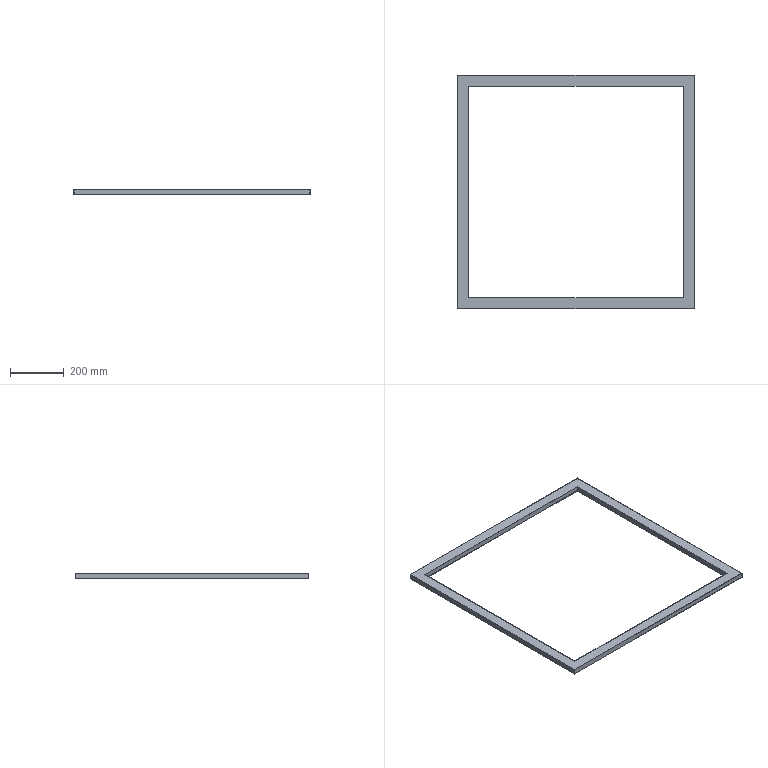Component | SolidWorks | 200TonPunchPress3DDrawing.sldasm-Part-1-1 | 1 solid | 20 faces | box 882 x 870 x 20 mm | volume 749056 mm3 | plane 20
STEP:
#1=COLOUR_RGB('',0.7922,0.8196,0.9333);
#2=FILL_AREA_STYLE_COLOUR('',#1);
#3=FILL_AREA_STYLE('',(#2));
#4=SURFACE_STYLE_FILL_AREA(#3);
#5=SURFACE_SIDE_STYLE('',(#4));
#6=SURFACE_STYLE_USAGE(.BOTH.,#5);
#7=PRESENTATION_STYLE_ASSIGNMENT((#6));
#8=CARTESIAN_POINT('',(-15.827,-41.278,51.26));
#9=VERTEX_POINT('',#8);
#10=CARTESIAN_POINT('',(15.906,-41.278,51.26));
#11=VERTEX_POINT('',#10);
#12=CARTESIAN_POINT('',(-20.057,-41.278,51.26));
#13=DIRECTION('',(1.,-0.,0.));
#14=VECTOR('',#13,39.37);
#15=LINE('',#12,#14);
#16=EDGE_CURVE('',#9,#11,#15,.T.);
#17=ORIENTED_EDGE('',*,*,#16,.T.);
#18=CARTESIAN_POINT('',(15.906,-41.278,51.89));
#19=VERTEX_POINT('',#18);
#20=CARTESIAN_POINT('',(15.906,-41.278,51.89));
#21=DIRECTION('',(0.,0.,1.));
#22=VECTOR('',#21,39.37);
#23=LINE('',#20,#22);
#24=EDGE_CURVE('',#11,#19,#23,.T.);
#25=ORIENTED_EDGE('',*,*,#24,.T.);
#26=CARTESIAN_POINT('',(-15.827,-41.278,51.89));
#27=VERTEX_POINT('',#26);
#28=CARTESIAN_POINT('',(-20.057,-41.278,51.89));
#29=DIRECTION('',(1.,-0.,0.));
#30=VECTOR('',#29,39.37);
#31=LINE('',#28,#30);
#32=EDGE_CURVE('',#27,#19,#31,.T.);
#33=ORIENTED_EDGE('',*,*,#32,.F.);
#34=CARTESIAN_POINT('',(-15.827,-41.278,51.89));
#35=DIRECTION('',(0.,0.,-1.));
#36=VECTOR('',#35,39.37);
#37=LINE('',#34,#36);
#38=EDGE_CURVE('',#27,#9,#37,.T.);
#39=ORIENTED_EDGE('',*,*,#38,.T.);
#40=EDGE_LOOP('',(#17,#25,#33,#39));
#41=FACE_OUTER_BOUND('',#40,.T.);
#42=CARTESIAN_POINT('',(-20.057,-41.278,51.89));
#43=DIRECTION('',(-0.,-1.,0.));
#44=DIRECTION('',(-1.,0.,0.));
#45=AXIS2_PLACEMENT_3D('',#42,#43,#44);
#46=PLANE('',#45);
#47=ADVANCED_FACE('',(#41),#46,.T.);
#48=CARTESIAN_POINT('',(15.906,-72.538,51.89));
#49=VERTEX_POINT('',#48);
#50=CARTESIAN_POINT('',(15.906,-72.538,51.89));
#51=DIRECTION('',(0.,1.,0.));
#52=VECTOR('',#51,39.37);
#53=LINE('',#50,#52);
#54=EDGE_CURVE('',#49,#19,#53,.T.);
#55=ORIENTED_EDGE('',*,*,#54,.F.);
#56=CARTESIAN_POINT('',(-15.827,-72.538,51.89));
#57=VERTEX_POINT('',#56);
#58=CARTESIAN_POINT('',(-15.827,-72.538,51.89));
#59=DIRECTION('',(1.,-0.,0.));
#60=VECTOR('',#59,39.37);
#61=LINE('',#58,#60);
#62=EDGE_CURVE('',#57,#49,#61,.T.);
#63=ORIENTED_EDGE('',*,*,#62,.F.);
#64=CARTESIAN_POINT('',(-15.827,-41.278,51.89));
#65=DIRECTION('',(0.,-1.,0.));
#66=VECTOR('',#65,39.37);
#67=LINE('',#64,#66);
#68=EDGE_CURVE('',#27,#57,#67,.T.);
#69=ORIENTED_EDGE('',*,*,#68,.F.);
#70=ORIENTED_EDGE('',*,*,#32,.T.);
#71=EDGE_LOOP('',(#55,#63,#69,#70));
#72=FACE_BOUND('',#71,.T.);
#73=CARTESIAN_POINT('',(-17.244,-73.955,51.89));
#74=VERTEX_POINT('',#73);
#75=CARTESIAN_POINT('',(17.323,-73.955,51.89));
#76=VERTEX_POINT('',#75);
#77=CARTESIAN_POINT('',(-17.244,-73.955,51.89));
#78=DIRECTION('',(1.,-0.,0.));
#79=VECTOR('',#78,39.37);
#80=LINE('',#77,#79);
#81=EDGE_CURVE('',#74,#76,#80,.T.);
#82=ORIENTED_EDGE('',*,*,#81,.T.);
#83=CARTESIAN_POINT('',(17.323,-39.86,51.89));
#84=VERTEX_POINT('',#83);
#85=CARTESIAN_POINT('',(17.323,-73.955,51.89));
#86=DIRECTION('',(0.,1.,0.));
#87=VECTOR('',#86,39.37);
#88=LINE('',#85,#87);
#89=EDGE_CURVE('',#76,#84,#88,.T.);
#90=ORIENTED_EDGE('',*,*,#89,.T.);
#91=CARTESIAN_POINT('',(-17.244,-39.86,51.89));
#92=VERTEX_POINT('',#91);
#93=CARTESIAN_POINT('',(-20.057,-39.86,51.89));
#94=DIRECTION('',(1.,-0.,0.));
#95=VECTOR('',#94,39.37);
#96=LINE('',#93,#95);
#97=EDGE_CURVE('',#92,#84,#96,.T.);
#98=ORIENTED_EDGE('',*,*,#97,.F.);
#99=CARTESIAN_POINT('',(-17.244,-39.86,51.89));
#100=DIRECTION('',(0.,-1.,0.));
#101=VECTOR('',#100,39.37);
#102=LINE('',#99,#101);
#103=EDGE_CURVE('',#92,#74,#102,.T.);
#104=ORIENTED_EDGE('',*,*,#103,.T.);
#105=EDGE_LOOP('',(#82,#90,#98,#104));
#106=FACE_OUTER_BOUND('',#105,.T.);
#107=CARTESIAN_POINT('',(-20.057,-39.86,51.89));
#108=DIRECTION('',(0.,0.,1.));
#109=DIRECTION('',(-1.,0.,0.));
#110=AXIS2_PLACEMENT_3D('',#107,#108,#109);
#111=PLANE('',#110);
#112=ADVANCED_FACE('',(#72,#106),#111,.T.);
#113=ORIENTED_EDGE('',*,*,#97,.T.);
#114=CARTESIAN_POINT('',(17.323,-39.86,51.26));
#115=VERTEX_POINT('',#114);
#116=CARTESIAN_POINT('',(17.323,-39.86,51.89));
#117=DIRECTION('',(0.,0.,-1.));
#118=VECTOR('',#117,39.37);
#119=LINE('',#116,#118);
#120=EDGE_CURVE('',#84,#115,#119,.T.);
#121=ORIENTED_EDGE('',*,*,#120,.T.);
#122=CARTESIAN_POINT('',(-17.244,-39.86,51.26));
#123=VERTEX_POINT('',#122);
#124=CARTESIAN_POINT('',(-20.057,-39.86,51.26));
#125=DIRECTION('',(1.,-0.,0.));
#126=VECTOR('',#125,39.37);
#127=LINE('',#124,#126);
#128=EDGE_CURVE('',#123,#115,#127,.T.);
#129=ORIENTED_EDGE('',*,*,#128,.F.);
#130=CARTESIAN_POINT('',(-17.244,-39.86,51.89));
#131=DIRECTION('',(0.,0.,1.));
#132=VECTOR('',#131,39.37);
#133=LINE('',#130,#132);
#134=EDGE_CURVE('',#123,#92,#133,.T.);
#135=ORIENTED_EDGE('',*,*,#134,.T.);
#136=EDGE_LOOP('',(#113,#121,#129,#135));
#137=FACE_OUTER_BOUND('',#136,.T.);
#138=CARTESIAN_POINT('',(-20.057,-39.86,51.89));
#139=DIRECTION('',(0.,1.,0.));
#140=DIRECTION('',(1.,-0.,0.));
#141=AXIS2_PLACEMENT_3D('',#138,#139,#140);
#142=PLANE('',#141);
#143=ADVANCED_FACE('',(#137),#142,.T.);
#144=CARTESIAN_POINT('',(17.323,-73.955,51.26));
#145=VERTEX_POINT('',#144);
#146=CARTESIAN_POINT('',(17.323,-73.955,51.89));
#147=DIRECTION('',(0.,0.,1.));
#148=VECTOR('',#147,39.37);
#149=LINE('',#146,#148);
#150=EDGE_CURVE('',#145,#76,#149,.T.);
#151=ORIENTED_EDGE('',*,*,#150,.F.);
#152=CARTESIAN_POINT('',(17.323,-73.955,51.26));
#153=DIRECTION('',(0.,1.,0.));
#154=VECTOR('',#153,39.37);
#155=LINE('',#152,#154);
#156=EDGE_CURVE('',#145,#115,#155,.T.);
#157=ORIENTED_EDGE('',*,*,#156,.T.);
#158=ORIENTED_EDGE('',*,*,#120,.F.);
#159=ORIENTED_EDGE('',*,*,#89,.F.);
#160=EDGE_LOOP('',(#151,#157,#158,#159));
#161=FACE_OUTER_BOUND('',#160,.T.);
#162=CARTESIAN_POINT('',(17.323,-73.955,51.89));
#163=DIRECTION('',(-1.,0.,0.));
#164=DIRECTION('',(0.,0.,-1.));
#165=AXIS2_PLACEMENT_3D('',#162,#163,#164);
#166=PLANE('',#165);
#167=ADVANCED_FACE('',(#161),#166,.F.);
#168=CARTESIAN_POINT('',(15.906,-72.538,51.26));
#169=VERTEX_POINT('',#168);
#170=CARTESIAN_POINT('',(15.906,-72.538,51.89));
#171=DIRECTION('',(0.,0.,-1.));
#172=VECTOR('',#171,39.37);
#173=LINE('',#170,#172);
#174=EDGE_CURVE('',#49,#169,#173,.T.);
#175=ORIENTED_EDGE('',*,*,#174,.F.);
#176=ORIENTED_EDGE('',*,*,#54,.T.);
#177=ORIENTED_EDGE('',*,*,#24,.F.);
#178=CARTESIAN_POINT('',(15.906,-72.538,51.26));
#179=DIRECTION('',(0.,1.,0.));
#180=VECTOR('',#179,39.37);
#181=LINE('',#178,#180);
#182=EDGE_CURVE('',#169,#11,#181,.T.);
#183=ORIENTED_EDGE('',*,*,#182,.F.);
#184=EDGE_LOOP('',(#175,#176,#177,#183));
#185=FACE_OUTER_BOUND('',#184,.T.);
#186=CARTESIAN_POINT('',(15.906,-72.538,51.89));
#187=DIRECTION('',(1.,0.,0.));
#188=DIRECTION('',(0.,0.,1.));
#189=AXIS2_PLACEMENT_3D('',#186,#187,#188);
#190=PLANE('',#189);
#191=ADVANCED_FACE('',(#185),#190,.F.);
#192=CARTESIAN_POINT('',(-15.827,-72.538,51.26));
#193=VERTEX_POINT('',#192);
#194=CARTESIAN_POINT('',(-15.827,-72.538,51.26));
#195=DIRECTION('',(1.,-0.,0.));
#196=VECTOR('',#195,39.37);
#197=LINE('',#194,#196);
#198=EDGE_CURVE('',#193,#169,#197,.T.);
#199=ORIENTED_EDGE('',*,*,#198,.F.);
#200=CARTESIAN_POINT('',(-15.827,-72.538,51.89));
#201=DIRECTION('',(0.,0.,1.));
#202=VECTOR('',#201,39.37);
#203=LINE('',#200,#202);
#204=EDGE_CURVE('',#193,#57,#203,.T.);
#205=ORIENTED_EDGE('',*,*,#204,.T.);
#206=ORIENTED_EDGE('',*,*,#62,.T.);
#207=ORIENTED_EDGE('',*,*,#174,.T.);
#208=EDGE_LOOP('',(#199,#205,#206,#207));
#209=FACE_OUTER_BOUND('',#208,.T.);
#210=CARTESIAN_POINT('',(-15.827,-72.538,51.89));
#211=DIRECTION('',(0.,1.,0.));
#212=DIRECTION('',(1.,-0.,0.));
#213=AXIS2_PLACEMENT_3D('',#210,#211,#212);
#214=PLANE('',#213);
#215=ADVANCED_FACE('',(#209),#214,.T.);
#216=ORIENTED_EDGE('',*,*,#38,.F.);
#217=ORIENTED_EDGE('',*,*,#68,.T.);
#218=ORIENTED_EDGE('',*,*,#204,.F.);
#219=CARTESIAN_POINT('',(-15.827,-41.278,51.26));
#220=DIRECTION('',(0.,-1.,0.));
#221=VECTOR('',#220,39.37);
#222=LINE('',#219,#221);
#223=EDGE_CURVE('',#9,#193,#222,.T.);
#224=ORIENTED_EDGE('',*,*,#223,.F.);
#225=EDGE_LOOP('',(#216,#217,#218,#224));
#226=FACE_OUTER_BOUND('',#225,.T.);
#227=CARTESIAN_POINT('',(-15.827,-41.278,51.89));
#228=DIRECTION('',(-1.,0.,0.));
#229=DIRECTION('',(0.,0.,-1.));
#230=AXIS2_PLACEMENT_3D('',#227,#228,#229);
#231=PLANE('',#230);
#232=ADVANCED_FACE('',(#226),#231,.F.);
#233=ORIENTED_EDGE('',*,*,#134,.F.);
#234=CARTESIAN_POINT('',(-17.244,-73.955,51.26));
#235=VERTEX_POINT('',#234);
#236=CARTESIAN_POINT('',(-17.244,-39.86,51.26));
#237=DIRECTION('',(0.,-1.,0.));
#238=VECTOR('',#237,39.37);
#239=LINE('',#236,#238);
#240=EDGE_CURVE('',#123,#235,#239,.T.);
#241=ORIENTED_EDGE('',*,*,#240,.T.);
#242=CARTESIAN_POINT('',(-17.244,-73.955,51.89));
#243=DIRECTION('',(0.,0.,-1.));
#244=VECTOR('',#243,39.37);
#245=LINE('',#242,#244);
#246=EDGE_CURVE('',#74,#235,#245,.T.);
#247=ORIENTED_EDGE('',*,*,#246,.F.);
#248=ORIENTED_EDGE('',*,*,#103,.F.);
#249=EDGE_LOOP('',(#233,#241,#247,#248));
#250=FACE_OUTER_BOUND('',#249,.T.);
#251=CARTESIAN_POINT('',(-17.244,-39.86,51.89));
#252=DIRECTION('',(1.,0.,0.));
#253=DIRECTION('',(0.,0.,1.));
#254=AXIS2_PLACEMENT_3D('',#251,#252,#253);
#255=PLANE('',#254);
#256=ADVANCED_FACE('',(#250),#255,.F.);
#257=ORIENTED_EDGE('',*,*,#81,.F.);
#258=ORIENTED_EDGE('',*,*,#246,.T.);
#259=CARTESIAN_POINT('',(-17.244,-73.955,51.26));
#260=DIRECTION('',(1.,-0.,0.));
#261=VECTOR('',#260,39.37);
#262=LINE('',#259,#261);
#263=EDGE_CURVE('',#235,#145,#262,.T.);
#264=ORIENTED_EDGE('',*,*,#263,.T.);
#265=ORIENTED_EDGE('',*,*,#150,.T.);
#266=EDGE_LOOP('',(#257,#258,#264,#265));
#267=FACE_OUTER_BOUND('',#266,.T.);
#268=CARTESIAN_POINT('',(-17.244,-73.955,51.89));
#269=DIRECTION('',(-0.,-1.,0.));
#270=DIRECTION('',(-1.,0.,0.));
#271=AXIS2_PLACEMENT_3D('',#268,#269,#270);
#272=PLANE('',#271);
#273=ADVANCED_FACE('',(#267),#272,.T.);
#274=ORIENTED_EDGE('',*,*,#156,.F.);
#275=ORIENTED_EDGE('',*,*,#263,.F.);
#276=ORIENTED_EDGE('',*,*,#240,.F.);
#277=ORIENTED_EDGE('',*,*,#128,.T.);
#278=EDGE_LOOP('',(#274,#275,#276,#277));
#279=FACE_OUTER_BOUND('',#278,.T.);
#280=ORIENTED_EDGE('',*,*,#198,.T.);
#281=ORIENTED_EDGE('',*,*,#182,.T.);
#282=ORIENTED_EDGE('',*,*,#16,.F.);
#283=ORIENTED_EDGE('',*,*,#223,.T.);
#284=EDGE_LOOP('',(#280,#281,#282,#283));
#285=FACE_BOUND('',#284,.T.);
#286=CARTESIAN_POINT('',(-20.057,-39.86,51.26));
#287=DIRECTION('',(0.,0.,-1.));
#288=DIRECTION('',(1.,0.,0.));
#289=AXIS2_PLACEMENT_3D('',#286,#287,#288);
#290=PLANE('',#289);
#291=ADVANCED_FACE('',(#279,#285),#290,.T.);
#292=CLOSED_SHELL('',(#47,#112,#143,#167,#191,#215,#232,#256,#273,#291));
#293=CARTESIAN_POINT('',(17.402,-39.782,51.969));
#294=VERTEX_POINT('',#293);
#295=CARTESIAN_POINT('',(17.402,-39.782,51.181));
#296=VERTEX_POINT('',#295);
#297=CARTESIAN_POINT('',(17.402,-39.782,51.969));
#298=DIRECTION('',(0.,0.,-1.));
#299=VECTOR('',#298,39.37);
#300=LINE('',#297,#299);
#301=EDGE_CURVE('',#294,#296,#300,.T.);
#302=ORIENTED_EDGE('',*,*,#301,.F.);
#303=CARTESIAN_POINT('',(17.402,-74.034,51.969));
#304=VERTEX_POINT('',#303);
#305=CARTESIAN_POINT('',(17.402,-74.034,51.969));
#306=DIRECTION('',(0.,1.,0.));
#307=VECTOR('',#306,39.37);
#308=LINE('',#305,#307);
#309=EDGE_CURVE('',#304,#294,#308,.T.);
#310=ORIENTED_EDGE('',*,*,#309,.F.);
#311=CARTESIAN_POINT('',(17.402,-74.034,51.181));
#312=VERTEX_POINT('',#311);
#313=CARTESIAN_POINT('',(17.402,-74.034,51.969));
#314=DIRECTION('',(0.,0.,1.));
#315=VECTOR('',#314,39.37);
#316=LINE('',#313,#315);
#317=EDGE_CURVE('',#312,#304,#316,.T.);
#318=ORIENTED_EDGE('',*,*,#317,.F.);
#319=CARTESIAN_POINT('',(17.402,-74.034,51.181));
#320=DIRECTION('',(0.,1.,0.));
#321=VECTOR('',#320,39.37);
#322=LINE('',#319,#321);
#323=EDGE_CURVE('',#312,#296,#322,.T.);
#324=ORIENTED_EDGE('',*,*,#323,.T.);
#325=EDGE_LOOP('',(#302,#310,#318,#324));
#326=FACE_OUTER_BOUND('',#325,.T.);
#327=CARTESIAN_POINT('',(17.402,-74.034,51.969));
#328=DIRECTION('',(-1.,0.,0.));
#329=DIRECTION('',(0.,0.,-1.));
#330=AXIS2_PLACEMENT_3D('',#327,#328,#329);
#331=PLANE('',#330);
#332=ADVANCED_FACE('',(#326),#331,.F.);
#333=CARTESIAN_POINT('',(15.827,-41.356,51.181));
#334=VERTEX_POINT('',#333);
#335=CARTESIAN_POINT('',(15.827,-41.356,51.969));
#336=VERTEX_POINT('',#335);
#337=CARTESIAN_POINT('',(15.827,-41.356,51.969));
#338=DIRECTION('',(0.,0.,1.));
#339=VECTOR('',#338,39.37);
#340=LINE('',#337,#339);
#341=EDGE_CURVE('',#334,#336,#340,.T.);
#342=ORIENTED_EDGE('',*,*,#341,.F.);
#343=CARTESIAN_POINT('',(15.827,-72.459,51.181));
#344=VERTEX_POINT('',#343);
#345=CARTESIAN_POINT('',(15.827,-72.459,51.181));
#346=DIRECTION('',(0.,1.,0.));
#347=VECTOR('',#346,39.37);
#348=LINE('',#345,#347);
#349=EDGE_CURVE('',#344,#334,#348,.T.);
#350=ORIENTED_EDGE('',*,*,#349,.F.);
#351=CARTESIAN_POINT('',(15.827,-72.459,51.969));
#352=VERTEX_POINT('',#351);
#353=CARTESIAN_POINT('',(15.827,-72.459,51.969));
#354=DIRECTION('',(0.,0.,-1.));
#355=VECTOR('',#354,39.37);
#356=LINE('',#353,#355);
#357=EDGE_CURVE('',#352,#344,#356,.T.);
#358=ORIENTED_EDGE('',*,*,#357,.F.);
#359=CARTESIAN_POINT('',(15.827,-72.459,51.969));
#360=DIRECTION('',(0.,1.,0.));
#361=VECTOR('',#360,39.37);
#362=LINE('',#359,#361);
#363=EDGE_CURVE('',#352,#336,#362,.T.);
#364=ORIENTED_EDGE('',*,*,#363,.T.);
#365=EDGE_LOOP('',(#342,#350,#358,#364));
#366=FACE_OUTER_BOUND('',#365,.T.);
#367=CARTESIAN_POINT('',(15.827,-72.459,51.969));
#368=DIRECTION('',(1.,0.,0.));
#369=DIRECTION('',(0.,0.,1.));
#370=AXIS2_PLACEMENT_3D('',#367,#368,#369);
#371=PLANE('',#370);
#372=ADVANCED_FACE('',(#366),#371,.F.);
#373=CARTESIAN_POINT('',(-17.323,-74.034,51.181));
#374=VERTEX_POINT('',#373);
#375=CARTESIAN_POINT('',(-17.323,-74.034,51.181));
#376=DIRECTION('',(1.,-0.,0.));
#377=VECTOR('',#376,39.37);
#378=LINE('',#375,#377);
#379=EDGE_CURVE('',#374,#312,#378,.T.);
#380=ORIENTED_EDGE('',*,*,#379,.T.);
#381=ORIENTED_EDGE('',*,*,#317,.T.);
#382=CARTESIAN_POINT('',(-17.323,-74.034,51.969));
#383=VERTEX_POINT('',#382);
#384=CARTESIAN_POINT('',(-17.323,-74.034,51.969));
#385=DIRECTION('',(1.,-0.,0.));
#386=VECTOR('',#385,39.37);
#387=LINE('',#384,#386);
#388=EDGE_CURVE('',#383,#304,#387,.T.);
#389=ORIENTED_EDGE('',*,*,#388,.F.);
#390=CARTESIAN_POINT('',(-17.323,-74.034,51.969));
#391=DIRECTION('',(0.,0.,-1.));
#392=VECTOR('',#391,39.37);
#393=LINE('',#390,#392);
#394=EDGE_CURVE('',#383,#374,#393,.T.);
#395=ORIENTED_EDGE('',*,*,#394,.T.);
#396=EDGE_LOOP('',(#380,#381,#389,#395));
#397=FACE_OUTER_BOUND('',#396,.T.);
#398=CARTESIAN_POINT('',(-17.323,-74.034,51.969));
#399=DIRECTION('',(-0.,-1.,0.));
#400=DIRECTION('',(-1.,0.,0.));
#401=AXIS2_PLACEMENT_3D('',#398,#399,#400);
#402=PLANE('',#401);
#403=ADVANCED_FACE('',(#397),#402,.T.);
#404=CARTESIAN_POINT('',(-15.748,-72.459,51.969));
#405=VERTEX_POINT('',#404);
#406=CARTESIAN_POINT('',(-15.748,-72.459,51.969));
#407=DIRECTION('',(1.,-0.,0.));
#408=VECTOR('',#407,39.37);
#409=LINE('',#406,#408);
#410=EDGE_CURVE('',#405,#352,#409,.T.);
#411=ORIENTED_EDGE('',*,*,#410,.T.);
#412=ORIENTED_EDGE('',*,*,#357,.T.);
#413=CARTESIAN_POINT('',(-15.748,-72.459,51.181));
#414=VERTEX_POINT('',#413);
#415=CARTESIAN_POINT('',(-15.748,-72.459,51.181));
#416=DIRECTION('',(1.,-0.,0.));
#417=VECTOR('',#416,39.37);
#418=LINE('',#415,#417);
#419=EDGE_CURVE('',#414,#344,#418,.T.);
#420=ORIENTED_EDGE('',*,*,#419,.F.);
#421=CARTESIAN_POINT('',(-15.748,-72.459,51.969));
#422=DIRECTION('',(0.,0.,1.));
#423=VECTOR('',#422,39.37);
#424=LINE('',#421,#423);
#425=EDGE_CURVE('',#414,#405,#424,.T.);
#426=ORIENTED_EDGE('',*,*,#425,.T.);
#427=EDGE_LOOP('',(#411,#412,#420,#426));
#428=FACE_OUTER_BOUND('',#427,.T.);
#429=CARTESIAN_POINT('',(-15.748,-72.459,51.969));
#430=DIRECTION('',(0.,1.,0.));
#431=DIRECTION('',(1.,-0.,0.));
#432=AXIS2_PLACEMENT_3D('',#429,#430,#431);
#433=PLANE('',#432);
#434=ADVANCED_FACE('',(#428),#433,.T.);
#435=ORIENTED_EDGE('',*,*,#394,.F.);
#436=CARTESIAN_POINT('',(-17.323,-39.782,51.969));
#437=VERTEX_POINT('',#436);
#438=CARTESIAN_POINT('',(-17.323,-39.782,51.969));
#439=DIRECTION('',(0.,-1.,0.));
#440=VECTOR('',#439,39.37);
#441=LINE('',#438,#440);
#442=EDGE_CURVE('',#437,#383,#441,.T.);
#443=ORIENTED_EDGE('',*,*,#442,.F.);
#444=CARTESIAN_POINT('',(-17.323,-39.782,51.181));
#445=VERTEX_POINT('',#444);
#446=CARTESIAN_POINT('',(-17.323,-39.782,51.969));
#447=DIRECTION('',(0.,0.,1.));
#448=VECTOR('',#447,39.37);
#449=LINE('',#446,#448);
#450=EDGE_CURVE('',#445,#437,#449,.T.);
#451=ORIENTED_EDGE('',*,*,#450,.F.);
#452=CARTESIAN_POINT('',(-17.323,-39.782,51.181));
#453=DIRECTION('',(0.,-1.,0.));
#454=VECTOR('',#453,39.37);
#455=LINE('',#452,#454);
#456=EDGE_CURVE('',#445,#374,#455,.T.);
#457=ORIENTED_EDGE('',*,*,#456,.T.);
#458=EDGE_LOOP('',(#435,#443,#451,#457));
#459=FACE_OUTER_BOUND('',#458,.T.);
#460=CARTESIAN_POINT('',(-17.323,-39.782,51.969));
#461=DIRECTION('',(1.,0.,0.));
#462=DIRECTION('',(0.,0.,1.));
#463=AXIS2_PLACEMENT_3D('',#460,#461,#462);
#464=PLANE('',#463);
#465=ADVANCED_FACE('',(#459),#464,.F.);
#466=ORIENTED_EDGE('',*,*,#425,.F.);
#467=CARTESIAN_POINT('',(-15.748,-41.356,51.181));
#468=VERTEX_POINT('',#467);
#469=CARTESIAN_POINT('',(-15.748,-41.356,51.181));
#470=DIRECTION('',(0.,-1.,0.));
#471=VECTOR('',#470,39.37);
#472=LINE('',#469,#471);
#473=EDGE_CURVE('',#468,#414,#472,.T.);
#474=ORIENTED_EDGE('',*,*,#473,.F.);
#475=CARTESIAN_POINT('',(-15.748,-41.356,51.969));
#476=VERTEX_POINT('',#475);
#477=CARTESIAN_POINT('',(-15.748,-41.356,51.969));
#478=DIRECTION('',(0.,0.,-1.));
#479=VECTOR('',#478,39.37);
#480=LINE('',#477,#479);
#481=EDGE_CURVE('',#476,#468,#480,.T.);
#482=ORIENTED_EDGE('',*,*,#481,.F.);
#483=CARTESIAN_POINT('',(-15.748,-41.356,51.969));
#484=DIRECTION('',(0.,-1.,0.));
#485=VECTOR('',#484,39.37);
#486=LINE('',#483,#485);
#487=EDGE_CURVE('',#476,#405,#486,.T.);
#488=ORIENTED_EDGE('',*,*,#487,.T.);
#489=EDGE_LOOP('',(#466,#474,#482,#488));
#490=FACE_OUTER_BOUND('',#489,.T.);
#491=CARTESIAN_POINT('',(-15.748,-41.356,51.969));
#492=DIRECTION('',(-1.,0.,0.));
#493=DIRECTION('',(0.,0.,-1.));
#494=AXIS2_PLACEMENT_3D('',#491,#492,#493);
#495=PLANE('',#494);
#496=ADVANCED_FACE('',(#490),#495,.F.);
#497=CARTESIAN_POINT('',(-20.057,-39.782,51.181));
#498=DIRECTION('',(1.,-0.,0.));
#499=VECTOR('',#498,39.37);
#500=LINE('',#497,#499);
#501=EDGE_CURVE('',#445,#296,#500,.T.);
#502=ORIENTED_EDGE('',*,*,#501,.F.);
#503=ORIENTED_EDGE('',*,*,#450,.T.);
#504=CARTESIAN_POINT('',(-20.057,-39.782,51.969));
#505=DIRECTION('',(1.,-0.,0.));
#506=VECTOR('',#505,39.37);
#507=LINE('',#504,#506);
#508=EDGE_CURVE('',#437,#294,#507,.T.);
#509=ORIENTED_EDGE('',*,*,#508,.T.);
#510=ORIENTED_EDGE('',*,*,#301,.T.);
#511=EDGE_LOOP('',(#502,#503,#509,#510));
#512=FACE_OUTER_BOUND('',#511,.T.);
#513=CARTESIAN_POINT('',(-20.057,-39.782,51.969));
#514=DIRECTION('',(0.,1.,0.));
#515=DIRECTION('',(1.,-0.,0.));
#516=AXIS2_PLACEMENT_3D('',#513,#514,#515);
#517=PLANE('',#516);
#518=ADVANCED_FACE('',(#512),#517,.T.);
#519=ORIENTED_EDGE('',*,*,#456,.F.);
#520=ORIENTED_EDGE('',*,*,#501,.T.);
#521=ORIENTED_EDGE('',*,*,#323,.F.);
#522=ORIENTED_EDGE('',*,*,#379,.F.);
#523=EDGE_LOOP('',(#519,#520,#521,#522));
#524=FACE_OUTER_BOUND('',#523,.T.);
#525=CARTESIAN_POINT('',(-20.057,-41.356,51.181));
#526=DIRECTION('',(1.,-0.,0.));
#527=VECTOR('',#526,39.37);
#528=LINE('',#525,#527);
#529=EDGE_CURVE('',#468,#334,#528,.T.);
#530=ORIENTED_EDGE('',*,*,#529,.F.);
#531=ORIENTED_EDGE('',*,*,#473,.T.);
#532=ORIENTED_EDGE('',*,*,#419,.T.);
#533=ORIENTED_EDGE('',*,*,#349,.T.);
#534=EDGE_LOOP('',(#530,#531,#532,#533));
#535=FACE_BOUND('',#534,.T.);
#536=CARTESIAN_POINT('',(-20.057,-39.782,51.181));
#537=DIRECTION('',(0.,0.,-1.));
#538=DIRECTION('',(0.,-1.,-0.));
#539=AXIS2_PLACEMENT_3D('',#536,#537,#538);
#540=PLANE('',#539);
#541=ADVANCED_FACE('',(#524,#535),#540,.T.);
#542=CARTESIAN_POINT('',(-20.057,-41.356,51.969));
#543=DIRECTION('',(1.,-0.,0.));
#544=VECTOR('',#543,39.37);
#545=LINE('',#542,#544);
#546=EDGE_CURVE('',#476,#336,#545,.T.);
#547=ORIENTED_EDGE('',*,*,#546,.F.);
#548=ORIENTED_EDGE('',*,*,#481,.T.);
#549=ORIENTED_EDGE('',*,*,#529,.T.);
#550=ORIENTED_EDGE('',*,*,#341,.T.);
#551=EDGE_LOOP('',(#547,#548,#549,#550));
#552=FACE_OUTER_BOUND('',#551,.T.);
#553=CARTESIAN_POINT('',(-20.057,-41.356,51.969));
#554=DIRECTION('',(-0.,-1.,0.));
#555=DIRECTION('',(-1.,0.,0.));
#556=AXIS2_PLACEMENT_3D('',#553,#554,#555);
#557=PLANE('',#556);
#558=ADVANCED_FACE('',(#552),#557,.T.);
#559=ORIENTED_EDGE('',*,*,#487,.F.);
#560=ORIENTED_EDGE('',*,*,#546,.T.);
#561=ORIENTED_EDGE('',*,*,#363,.F.);
#562=ORIENTED_EDGE('',*,*,#410,.F.);
#563=EDGE_LOOP('',(#559,#560,#561,#562));
#564=FACE_BOUND('',#563,.T.);
#565=ORIENTED_EDGE('',*,*,#508,.F.);
#566=ORIENTED_EDGE('',*,*,#442,.T.);
#567=ORIENTED_EDGE('',*,*,#388,.T.);
#568=ORIENTED_EDGE('',*,*,#309,.T.);
#569=EDGE_LOOP('',(#565,#566,#567,#568));
#570=FACE_OUTER_BOUND('',#569,.T.);
#571=CARTESIAN_POINT('',(-20.057,-39.782,51.969));
#572=DIRECTION('',(-0.,-0.,1.));
#573=DIRECTION('',(0.,1.,0.));
#574=AXIS2_PLACEMENT_3D('',#571,#572,#573);
#575=PLANE('',#574);
#576=ADVANCED_FACE('',(#564,#570),#575,.T.);
#577=CLOSED_SHELL('',(#332,#372,#403,#434,#465,#496,#518,#541,#558,#576));
#578=ORIENTED_CLOSED_SHELL('',*,#577,.F.);
#579=BREP_WITH_VOIDS('',#292,(#578));
#580=STYLED_ITEM('',(#7),#579);
#581=PRESENTATION_LAYER_ASSIGNMENT('','',(#580));
#582=(LENGTH_UNIT()NAMED_UNIT(*)SI_UNIT($,.METRE.));
#583=LENGTH_MEASURE_WITH_UNIT(LENGTH_MEASURE(0.0254),#582);
#584=DIMENSIONAL_EXPONENTS(1.,0.,0.,0.,0.,0.,0.);
#585=(CONVERSION_BASED_UNIT('',#583)LENGTH_UNIT()NAMED_UNIT(#584));
#586=UNCERTAINTY_MEASURE_WITH_UNIT(LENGTH_MEASURE(0.00001),#585,'','');
#587=(NAMED_UNIT(*)PLANE_ANGLE_UNIT()SI_UNIT($,.RADIAN.));
#588=(NAMED_UNIT(*)SI_UNIT($,.STERADIAN.)SOLID_ANGLE_UNIT());
#589=(GEOMETRIC_REPRESENTATION_CONTEXT(3)GLOBAL_UNCERTAINTY_ASSIGNED_CONTEXT((#586))GLOBAL_UNIT_ASSIGNED_CONTEXT((#585,#587,#588))REPRESENTATION_CONTEXT('',''));
#590=MECHANICAL_DESIGN_GEOMETRIC_PRESENTATION_REPRESENTATION('',(#580),#589);
#591=CARTESIAN_POINT('',(0.,0.,0.));
#592=DIRECTION('',(0.,0.,1.));
#593=DIRECTION('',(1.,0.,0.));
#594=AXIS2_PLACEMENT_3D('',#591,#592,#593);
#595=(LENGTH_UNIT()NAMED_UNIT(*)SI_UNIT($,.METRE.));
#596=LENGTH_MEASURE_WITH_UNIT(LENGTH_MEASURE(0.0254),#595);
#597=DIMENSIONAL_EXPONENTS(1.,0.,0.,0.,0.,0.,0.);
#598=(CONVERSION_BASED_UNIT('',#596)LENGTH_UNIT()NAMED_UNIT(#597));
#599=UNCERTAINTY_MEASURE_WITH_UNIT(LENGTH_MEASURE(0.00001),#598,'','');
#600=(NAMED_UNIT(*)PLANE_ANGLE_UNIT()SI_UNIT($,.RADIAN.));
#601=(NAMED_UNIT(*)SI_UNIT($,.STERADIAN.)SOLID_ANGLE_UNIT());
#602=(GEOMETRIC_REPRESENTATION_CONTEXT(3)GLOBAL_UNCERTAINTY_ASSIGNED_CONTEXT((#599))GLOBAL_UNIT_ASSIGNED_CONTEXT((#598,#600,#601))REPRESENTATION_CONTEXT('',''));
#603=ADVANCED_BREP_SHAPE_REPRESENTATION('',(#579,#594),#602);